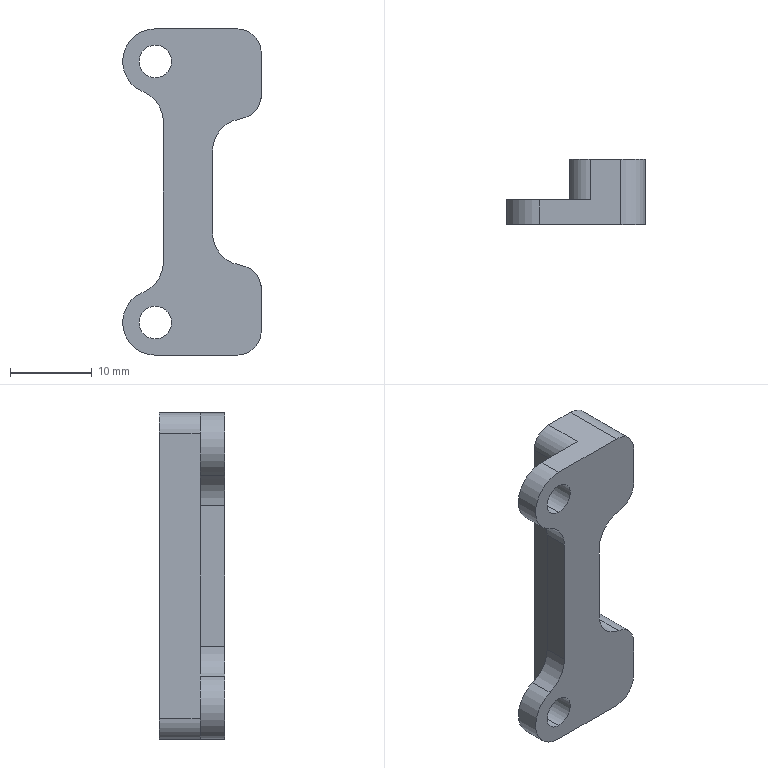CAM job | Mastercam | mm | 7 operations | part box 17 x 8 x 40
1. Facing | 24 - 100 平铣刀
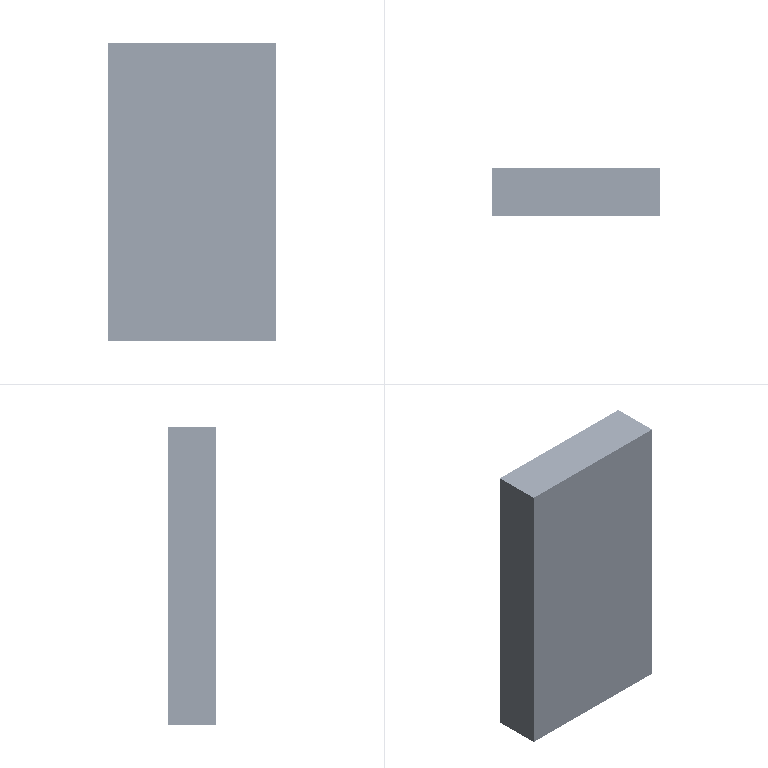2. 2D High Speed (2D Dynamic Mill) | 8 - 8 平铣刀
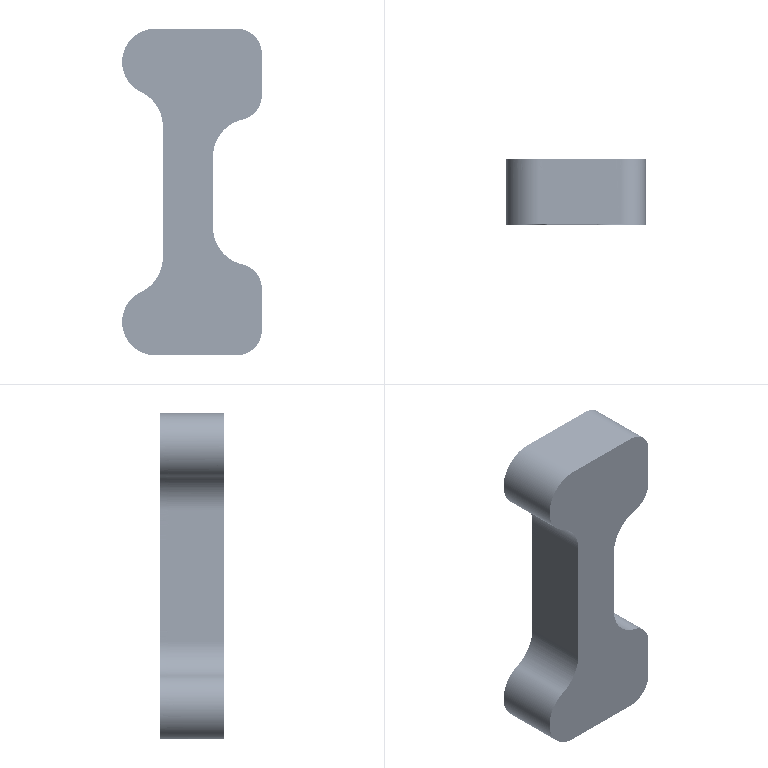3. Contour (Ramp) | 8 - 8 平铣刀
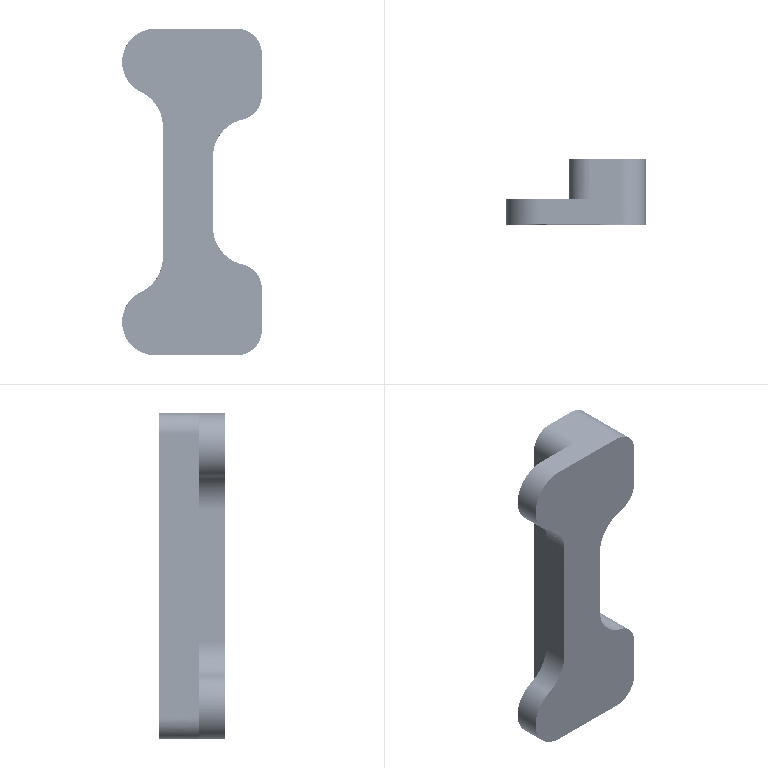4. Contour (2D) | 8 - 8 平铣刀
5. Contour (2D) | 8 - 8 平铣刀
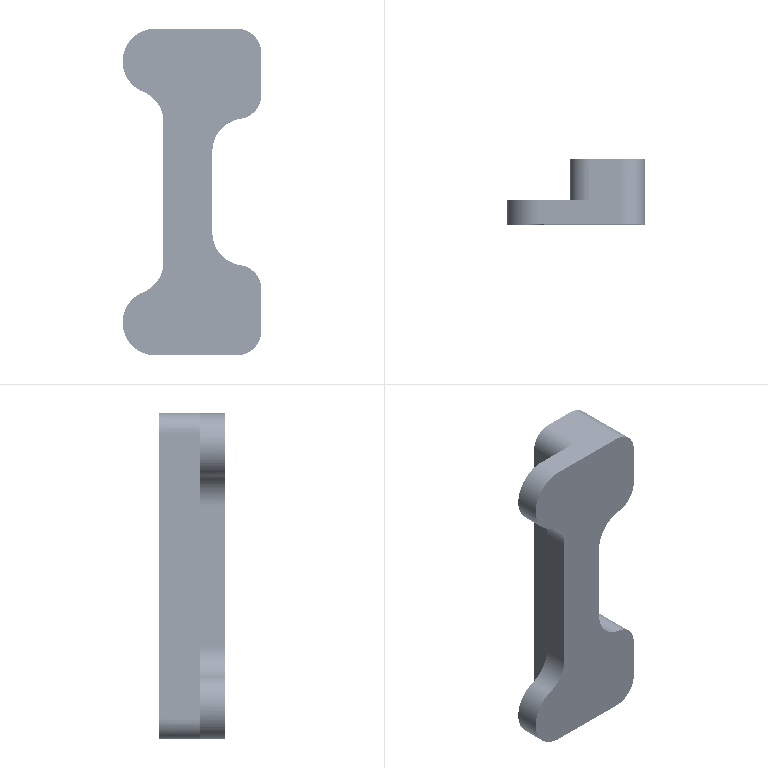6. Drill/Counterbore | 7 - 4 倒角刀
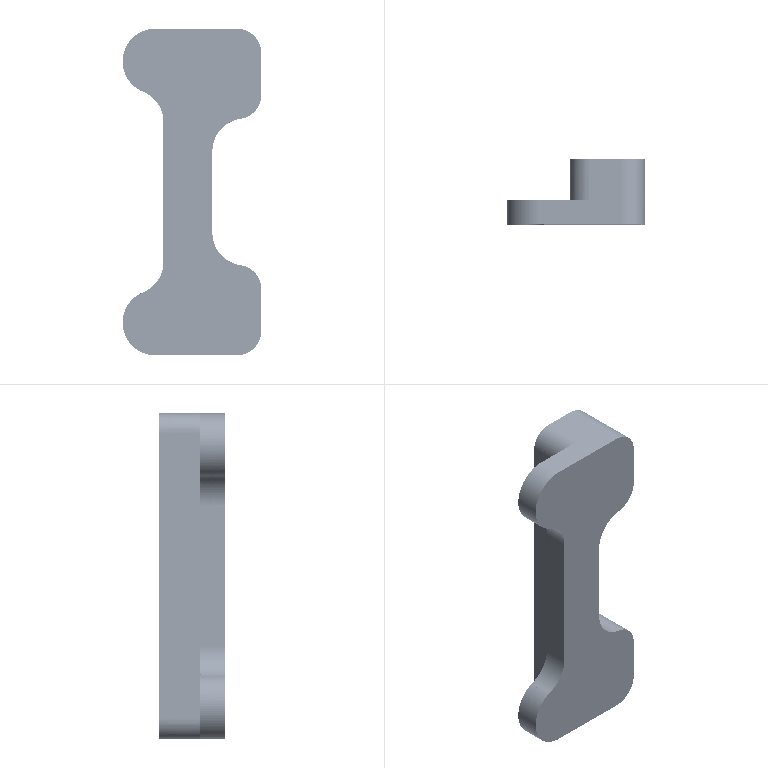7. Deburr 5-axis | 7 - 4 倒角刀